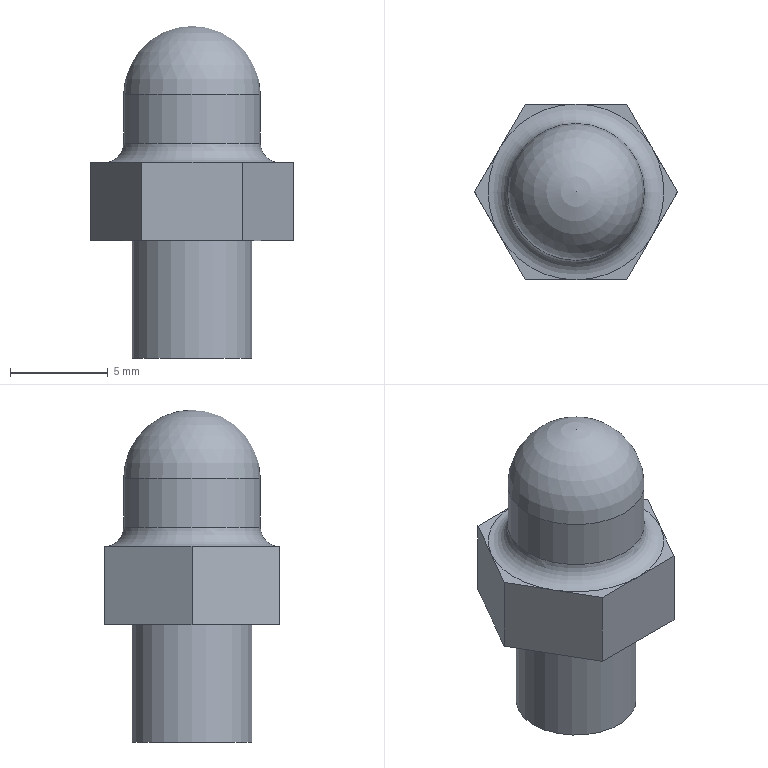Component | NX | UPPER_CONNECTING_NUT | 1 solid | 20 faces | volume 589 mm3 | plane 15 | cylinder 3 | sphere 1 | torus 1 | commonest cylinder face diameters 6.144 x1 7 x1 3 x1